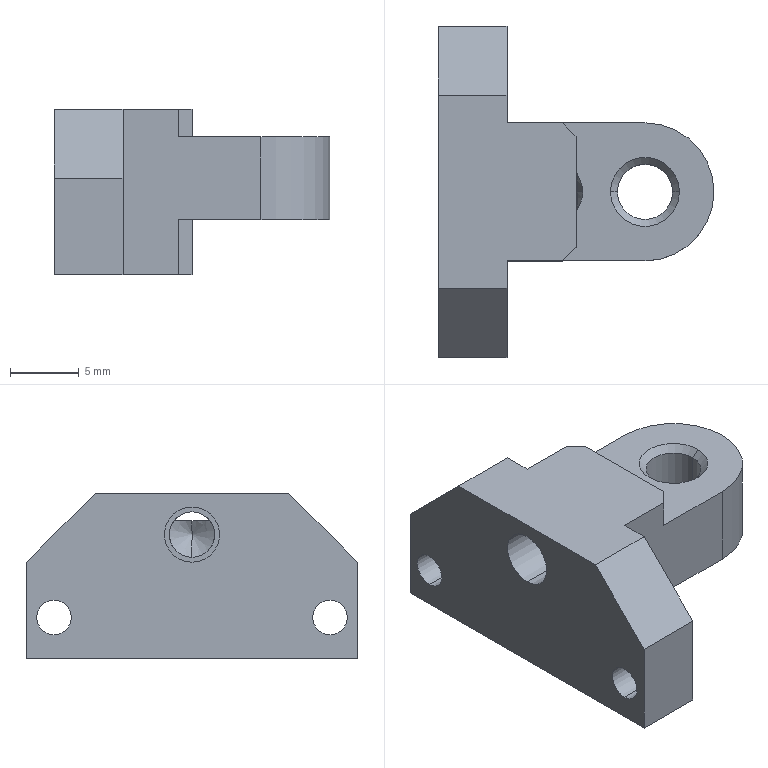Component | SolidWorks | JR-PL-JD-14FloatingHead-1 | 1 solid | 41 faces | box 20 x 24 x 12 mm | volume 2195 mm3 | plane 20 | cylinder 11 | cone 10 | commonest cylinder face diameters 4 x4 2.5 x4 3.3 x2 10 x1
build123d program:
from build123d import *

# Parameters (mm, degrees)
BOSS_EXTRUDE1_DEPTH              = 6
M4_TAPPED_HOLE1_D                = 3.3
M4_TAPPED_HOLE1_DEPTH            = 10.1
M4_TAPPED_HOLE1_TIP              = 0.9914
SIZE_MM_DOWEL_PIN_HOLE_1_D       = 4
SKETCH6_W                        = 10
SKETCH6_H                        = 2
SKETCH6_H_2                      = 4
CUT_EXTRUDE1_DEPTH               = 27.926
CHAMFER1_SIZE                    = 5
M3_TAPPED_HOLE1_D                = 2.5
M3_TAPPED_HOLE1_CSINK_D          = 3.05
M3_TAPPED_HOLE1_CSINK_ANGLE      = 90
CHAMFER2_SIZE                    = 1
CHAMFER3_SIZE                    = 0.5
SKETCH1_R                        = 2
M4_THREAD_MAJOR_DIA_RELIEF_DEPTH = 8


with BuildPart() as part:
    # Sketch1_2 → Boss-Extrude1 (new, symmetric)
    with BuildSketch(Plane.XY):
        with BuildLine():
            Line((15, 5), (5, 5))
            Line((5, 5), (5, 12))
            Line((5, 12), (0, 12))
            Line((0, 12), (0, -12))
            Line((0, -12), (5, -12))
            Line((5, -12), (5, -5))
            Line((5, -5), (15, -5))
            ThreePointArc((15, -5), (20, 0), (15, 5))
        make_face()
    extrude(amount=BOSS_EXTRUDE1_DEPTH, both=True)

    # M4 Tapped Hole1
    with Locations(Plane.ZY):
        with Locations((3, 0)):
            Hole(M4_TAPPED_HOLE1_D / 2, depth=M4_TAPPED_HOLE1_DEPTH)
            with Locations((0, 0, -(M4_TAPPED_HOLE1_DEPTH + M4_TAPPED_HOLE1_TIP / 2))):  # 118° drill point
                Cone(0, M4_TAPPED_HOLE1_D / 2, M4_TAPPED_HOLE1_TIP, mode=Mode.SUBTRACT)

    # Size mm Dowel Pin Hole 1 (through all)
    with Locations(Plane.XY.offset(6)):
        with Locations((15, 0)):
            Hole(SIZE_MM_DOWEL_PIN_HOLE_1_D / 2)

    # Sketch6 → Cut-Extrude1 (cut, through all)
    with BuildSketch(Plane.XZ.offset(5)):
        with Locations((15, 5)):
            Rectangle(SKETCH6_W, SKETCH6_H)
        with Locations((15, -4)):
            Rectangle(SKETCH6_W, SKETCH6_H_2)
    extrude(amount=-CUT_EXTRUDE1_DEPTH, mode=Mode.SUBTRACT)

    # Chamfer1
    chamfer1_edges = [part.edges().sort_by_distance(p)[0] for p in [
        (2.5, 12, 6),
        (2.5, -12, 6),
    ]]
    chamfer(chamfer1_edges, length=CHAMFER1_SIZE)

    # M3 Tapped Hole1 (through all)
    with Locations(Plane(origin=(5, 0, 0), x_dir=(0, 0, -1), z_dir=(1, 0, 0))):
        with Locations((3, -10), (3, 10)):
            CounterSinkHole(M3_TAPPED_HOLE1_D / 2, M3_TAPPED_HOLE1_CSINK_D / 2, counter_sink_angle=M3_TAPPED_HOLE1_CSINK_ANGLE)

    # Chamfer2
    chamfer2_edges = [part.edges().sort_by_distance(p)[0] for p in [
        (10, -5, 5),
        (10, 5, 5),
        (10, 5, -4),
        (10, -5, -4),
    ]]
    chamfer(chamfer2_edges, length=CHAMFER2_SIZE)

    # Chamfer3
    chamfer3_edges = [part.edges().sort_by_distance(p)[0] for p in [
        (17, 0, 4),
        (17, 0, -2),
    ]]
    chamfer(chamfer3_edges, length=CHAMFER3_SIZE)

    # Sketch1 → M4 thread major-dia relief (cut)
    with BuildSketch(Plane.ZY):
        with Locations((3, 0)):
            Circle(SKETCH1_R)
    extrude(amount=-M4_THREAD_MAJOR_DIA_RELIEF_DEPTH, mode=Mode.SUBTRACT)


solid = part.part

# Placed as in the assembly
solid = solid.moved(Location((1.506, 30.452, 69.77), (0, 0, 0)))